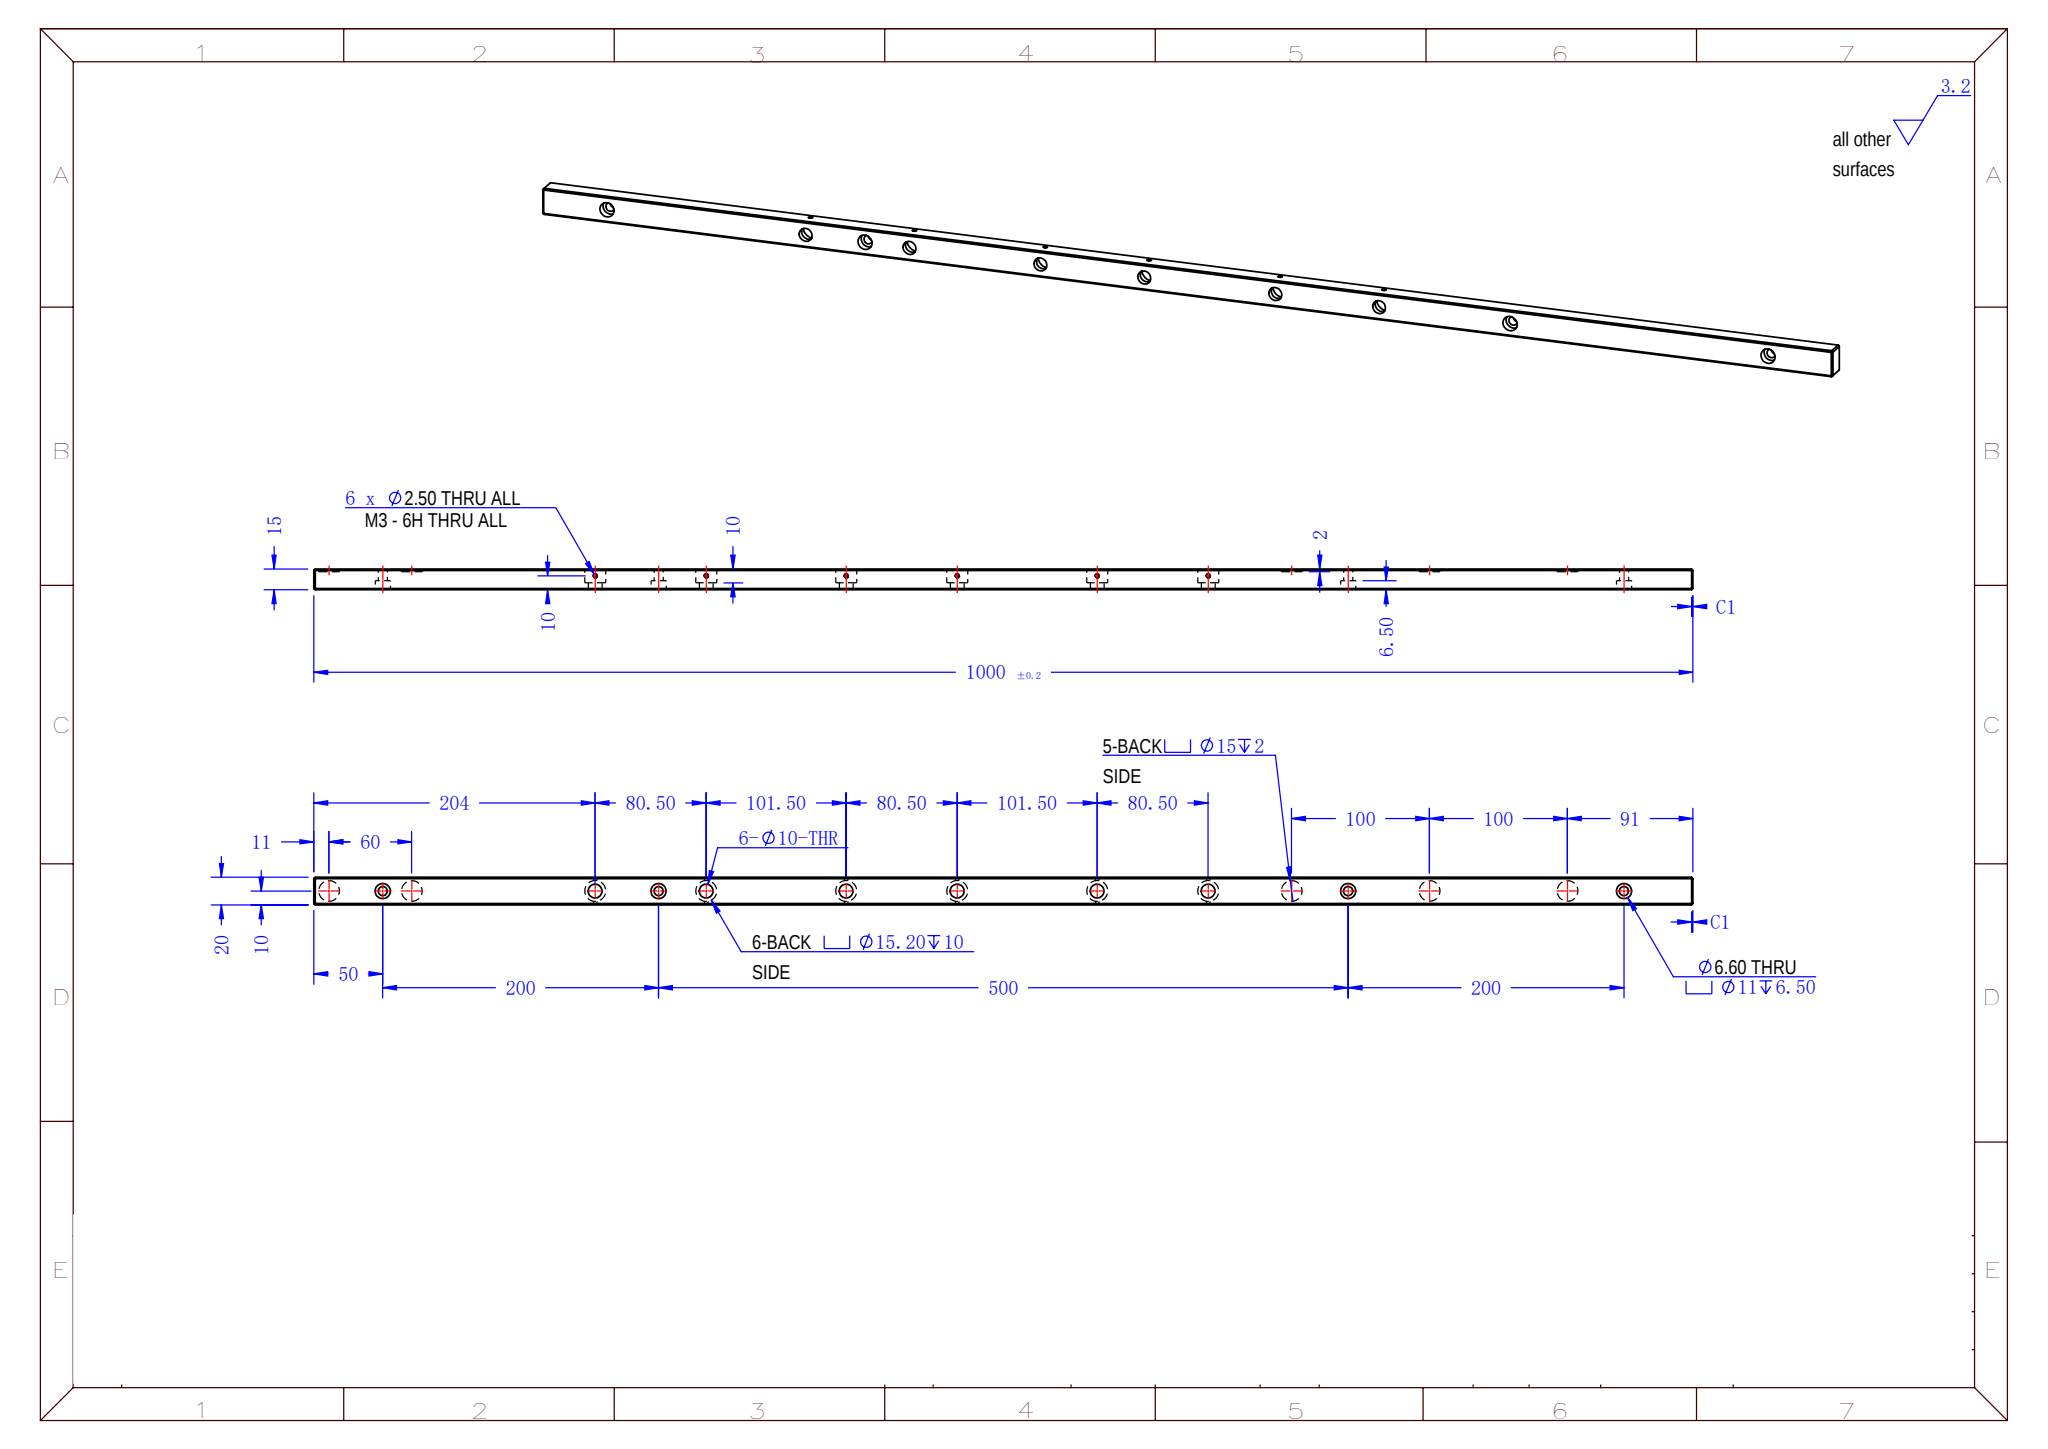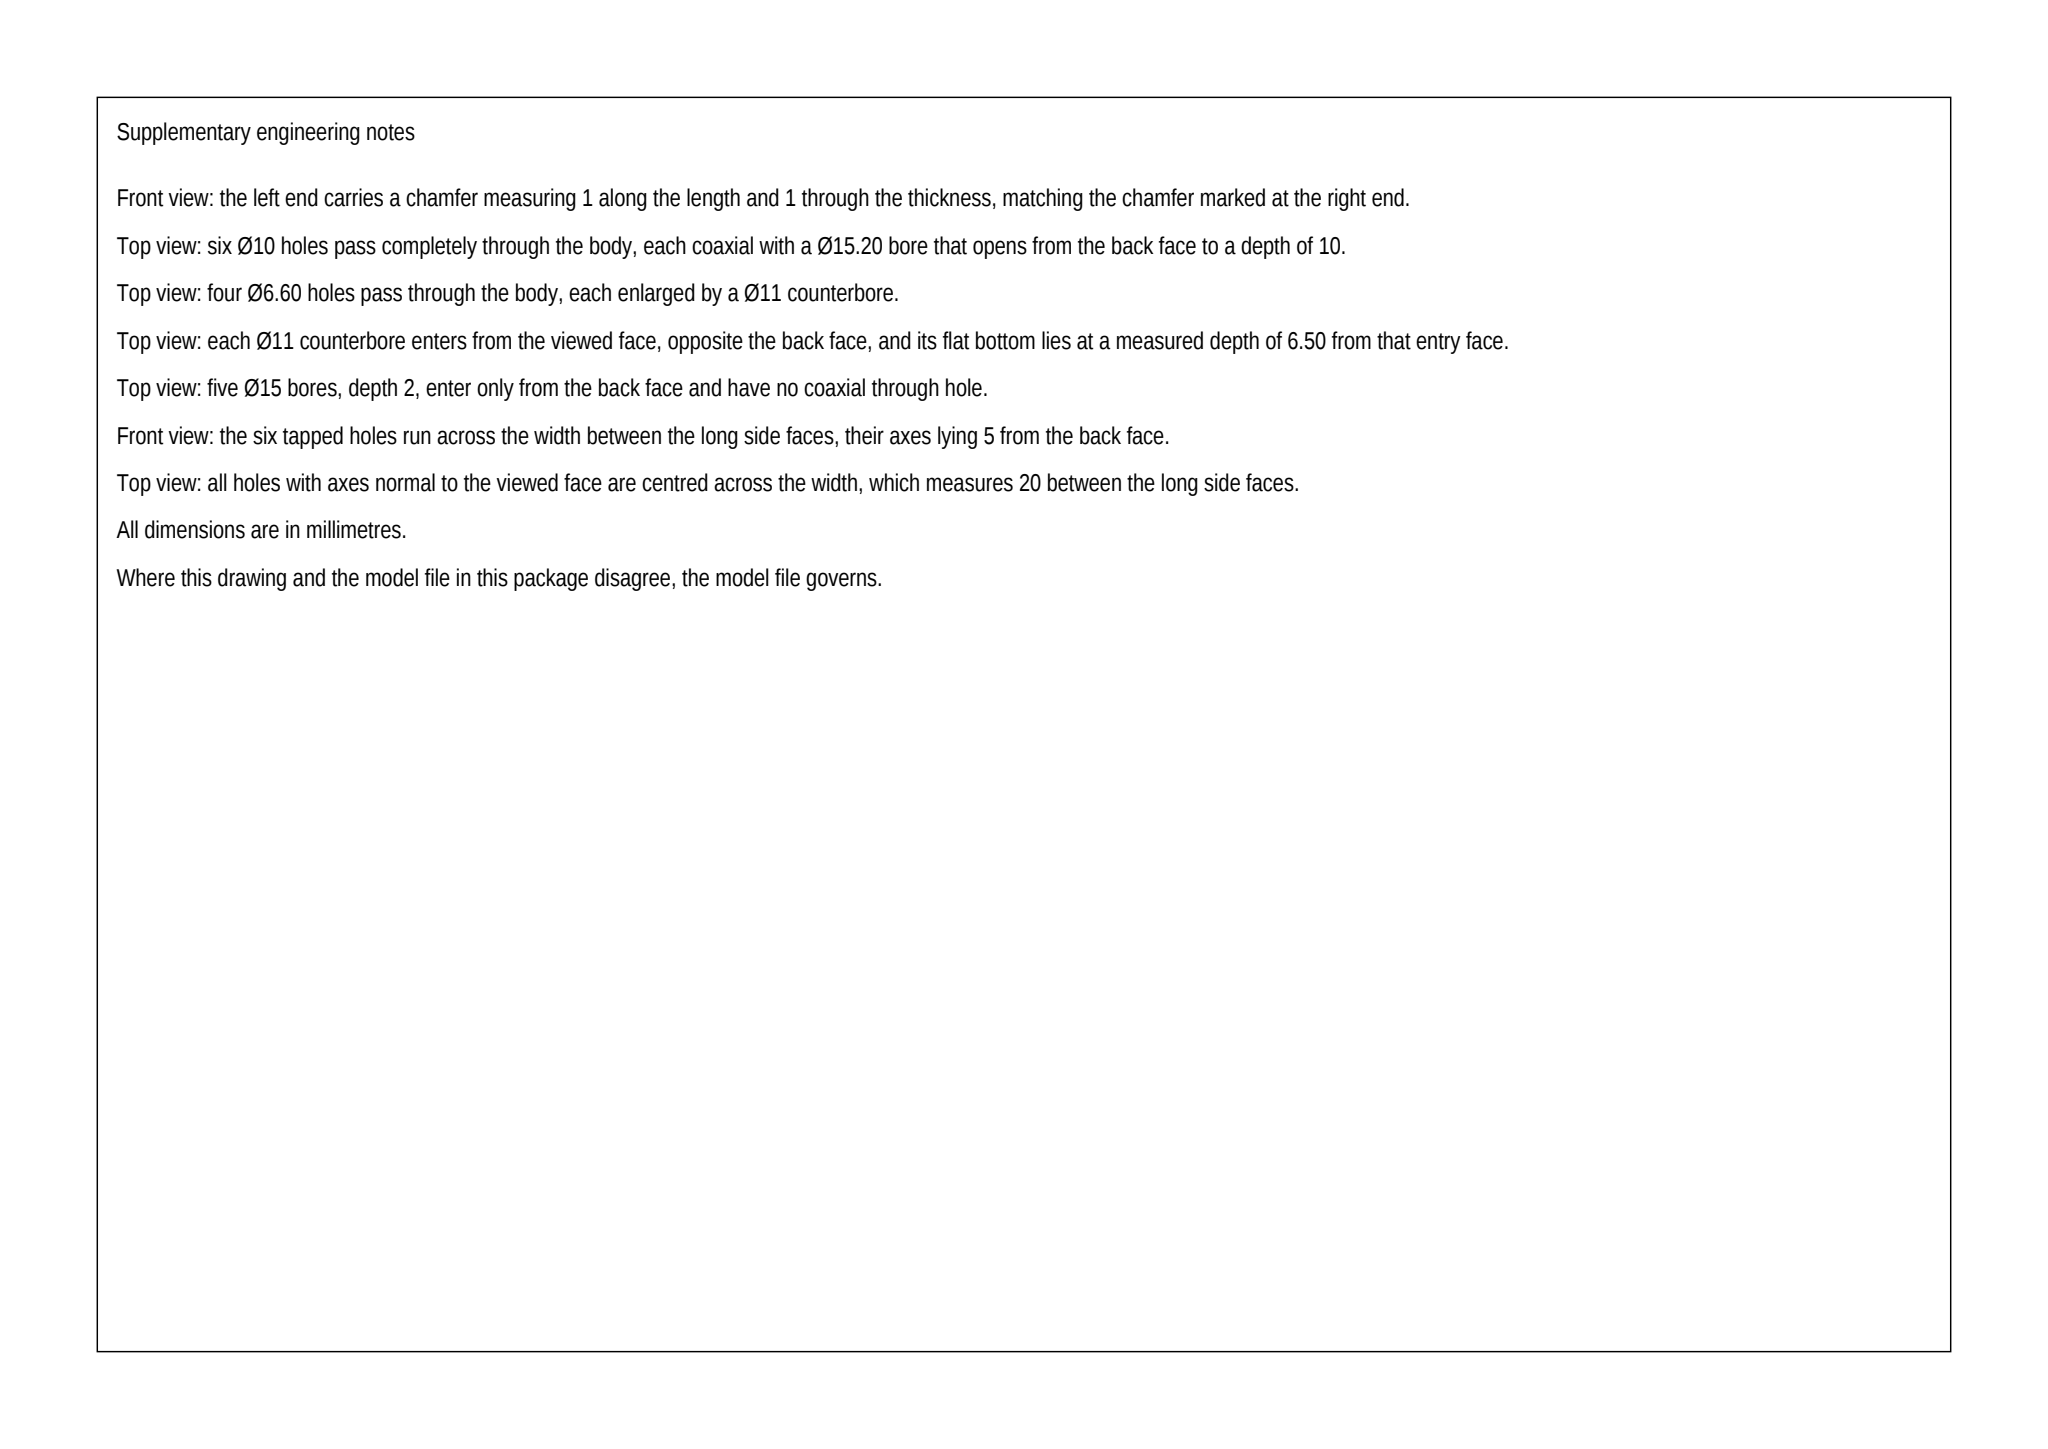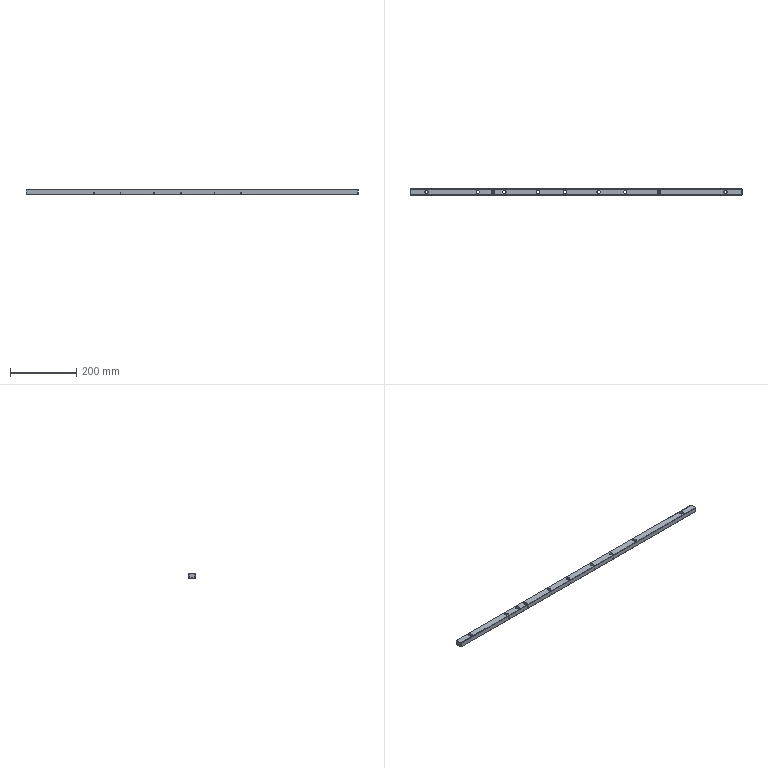Part | SolidWorks | mm | 1 solid | 107 faces | box 1000 x 20 x 15 mm | volume 279148 mm3 | cylinder 74 | plane 33 | commonest cylinder face diameters 2.5 x24 15.2 x12 10 x12 15 x10 11 x8 6.6 x8